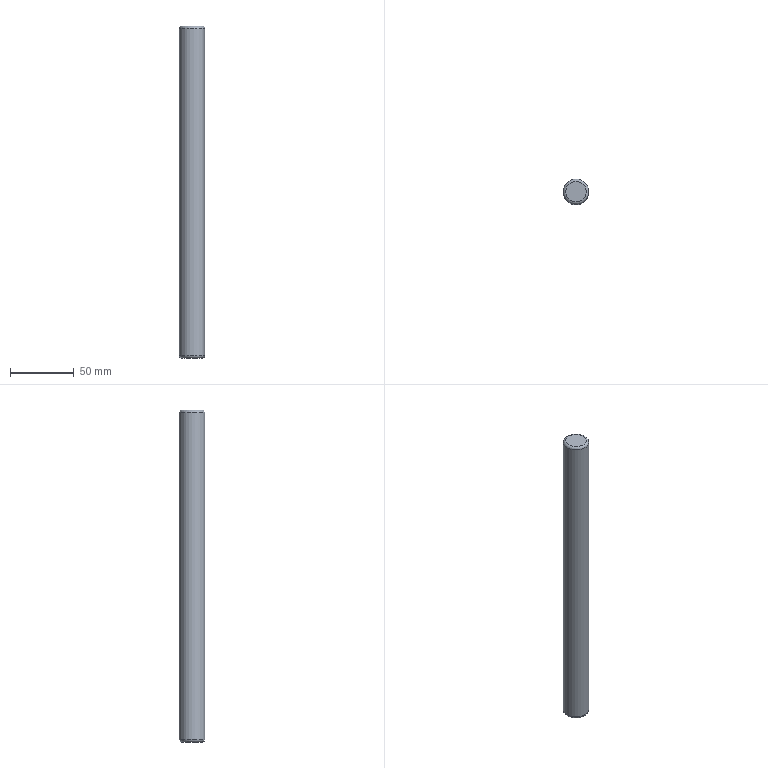Component | NX | CIBIK5 | 1 solid | 5 faces | box 20 x 20 x 260 mm | volume 81578 mm3 | plane 2 | torus 2 | cylinder 1 | commonest cylinder face diameters 20 x1
STEP:
#1=CARTESIAN_POINT('',(0.,0.,0.));
#2=DIRECTION('',(0.,0.,1.));
#3=DIRECTION('',(1.,0.,0.));
#4=AXIS2_PLACEMENT_3D('',#1,#2,#3);
#5=CARTESIAN_POINT('',(-1165.866,976.821,260.));
#6=VERTEX_POINT('',#5);
#7=CARTESIAN_POINT('',(-1155.866,976.821,260.));
#8=DIRECTION('',(0.,0.,-1.));
#9=DIRECTION('',(-1.,0.,0.));
#10=AXIS2_PLACEMENT_3D('',#7,#8,#9);
#11=CIRCLE('',#10,10.);
#12=CARTESIAN_POINT('',(-1155.866,976.821,2.));
#13=DIRECTION('',(0.,0.,1.));
#14=DIRECTION('',(1.,0.,0.));
#15=AXIS2_PLACEMENT_3D('',#12,#13,#14);
#16=CYLINDRICAL_SURFACE('',#15,10.);
#17=CARTESIAN_POINT('',(9.425,258.));
#18=DIRECTION('',(-1.,0.));
#19=VECTOR('',#18,1.);
#20=LINE('',#17,#19);
#21=(GEOMETRIC_REPRESENTATION_CONTEXT(2)PARAMETRIC_REPRESENTATION_CONTEXT()REPRESENTATION_CONTEXT('',''));
#22=DEFINITIONAL_REPRESENTATION('',(#20),#21);
#23=PCURVE('',#16,#22);
#24=CARTESIAN_POINT('',(-1155.866,976.821,260.));
#25=DIRECTION('',(0.,0.,-1.));
#26=DIRECTION('',(-1.,0.,0.));
#27=AXIS2_PLACEMENT_3D('',#24,#25,#26);
#28=TOROIDAL_SURFACE('',#27,8.,2.);
#29=CARTESIAN_POINT('',(0.,6.283));
#30=DIRECTION('',(1.,0.));
#31=VECTOR('',#30,1.);
#32=LINE('',#29,#31);
#33=(GEOMETRIC_REPRESENTATION_CONTEXT(2)PARAMETRIC_REPRESENTATION_CONTEXT()REPRESENTATION_CONTEXT('',''));
#34=DEFINITIONAL_REPRESENTATION('',(#32),#33);
#35=PCURVE('',#28,#34);
#36=SURFACE_CURVE('',#11,(#23,#35),.PCURVE_S1.);
#37=EDGE_CURVE('',#6,#6,#36,.T.);
#38=ORIENTED_EDGE('',*,*,#37,.T.);
#39=CARTESIAN_POINT('',(-1165.866,976.821,4.));
#40=VERTEX_POINT('',#39);
#41=CARTESIAN_POINT('',(-1165.866,976.821,4.));
#42=CARTESIAN_POINT('',(-1165.866,976.821,260.));
#43=B_SPLINE_CURVE_WITH_KNOTS('',1,(#41,#42),.UNSPECIFIED.,.F.,.F.,(2,2),(2.,258.),.PIECEWISE_BEZIER_KNOTS.);
#44=CARTESIAN_POINT('',(3.142,0.));
#45=DIRECTION('',(0.,1.));
#46=VECTOR('',#45,1.);
#47=LINE('',#44,#46);
#48=(GEOMETRIC_REPRESENTATION_CONTEXT(2)PARAMETRIC_REPRESENTATION_CONTEXT()REPRESENTATION_CONTEXT('',''));
#49=DEFINITIONAL_REPRESENTATION('',(#47),#48);
#50=PCURVE('',#16,#49);
#51=CARTESIAN_POINT('',(9.425,0.));
#52=DIRECTION('',(0.,1.));
#53=VECTOR('',#52,1.);
#54=LINE('',#51,#53);
#55=(GEOMETRIC_REPRESENTATION_CONTEXT(2)PARAMETRIC_REPRESENTATION_CONTEXT()REPRESENTATION_CONTEXT('',''));
#56=DEFINITIONAL_REPRESENTATION('',(#54),#55);
#57=PCURVE('',#16,#56);
#58=SEAM_CURVE('',#43,(#50,#57),.PCURVE_S1.);
#59=EDGE_CURVE('',#40,#6,#58,.T.);
#60=ORIENTED_EDGE('',*,*,#59,.F.);
#61=CARTESIAN_POINT('',(-1155.866,976.821,4.));
#62=DIRECTION('',(0.,0.,1.));
#63=DIRECTION('',(-1.,0.,0.));
#64=AXIS2_PLACEMENT_3D('',#61,#62,#63);
#65=CIRCLE('',#64,10.);
#66=CARTESIAN_POINT('',(3.142,2.));
#67=DIRECTION('',(1.,0.));
#68=VECTOR('',#67,1.);
#69=LINE('',#66,#68);
#70=(GEOMETRIC_REPRESENTATION_CONTEXT(2)PARAMETRIC_REPRESENTATION_CONTEXT()REPRESENTATION_CONTEXT('',''));
#71=DEFINITIONAL_REPRESENTATION('',(#69),#70);
#72=PCURVE('',#16,#71);
#73=CARTESIAN_POINT('',(-1155.866,976.821,4.));
#74=DIRECTION('',(0.,0.,-1.));
#75=DIRECTION('',(-1.,0.,0.));
#76=AXIS2_PLACEMENT_3D('',#73,#74,#75);
#77=TOROIDAL_SURFACE('',#76,8.,2.);
#78=CARTESIAN_POINT('',(6.283,6.283));
#79=DIRECTION('',(-1.,0.));
#80=VECTOR('',#79,1.);
#81=LINE('',#78,#80);
#82=(GEOMETRIC_REPRESENTATION_CONTEXT(2)PARAMETRIC_REPRESENTATION_CONTEXT()REPRESENTATION_CONTEXT('',''));
#83=DEFINITIONAL_REPRESENTATION('',(#81),#82);
#84=PCURVE('',#77,#83);
#85=SURFACE_CURVE('',#65,(#72,#84),.PCURVE_S1.);
#86=EDGE_CURVE('',#40,#40,#85,.T.);
#87=ORIENTED_EDGE('',*,*,#86,.T.);
#88=ORIENTED_EDGE('',*,*,#59,.T.);
#89=EDGE_LOOP('',(#38,#60,#87,#88));
#90=FACE_BOUND('',#89,.T.);
#91=ADVANCED_FACE('',(#90),#16,.T.);
#92=CARTESIAN_POINT('',(-1163.866,976.821,2.));
#93=VERTEX_POINT('',#92);
#94=CARTESIAN_POINT('',(-1155.866,976.821,2.));
#95=DIRECTION('',(0.,0.,-1.));
#96=DIRECTION('',(-1.,0.,0.));
#97=AXIS2_PLACEMENT_3D('',#94,#95,#96);
#98=CIRCLE('',#97,8.);
#99=CARTESIAN_POINT('',(-1155.866,976.821,2.));
#100=DIRECTION('',(0.,0.,-1.));
#101=DIRECTION('',(-1.,0.,0.));
#102=AXIS2_PLACEMENT_3D('',#99,#100,#101);
#103=PLANE('',#102);
#104=CARTESIAN_POINT('',(0.,0.));
#105=DIRECTION('',(1.,0.));
#106=AXIS2_PLACEMENT_2D('',#104,#105);
#107=CIRCLE('',#106,8.);
#108=(GEOMETRIC_REPRESENTATION_CONTEXT(2)PARAMETRIC_REPRESENTATION_CONTEXT()REPRESENTATION_CONTEXT('',''));
#109=DEFINITIONAL_REPRESENTATION('',(#107),#108);
#110=PCURVE('',#103,#109);
#111=CARTESIAN_POINT('',(0.,7.854));
#112=DIRECTION('',(1.,0.));
#113=VECTOR('',#112,1.);
#114=LINE('',#111,#113);
#115=(GEOMETRIC_REPRESENTATION_CONTEXT(2)PARAMETRIC_REPRESENTATION_CONTEXT()REPRESENTATION_CONTEXT('',''));
#116=DEFINITIONAL_REPRESENTATION('',(#114),#115);
#117=PCURVE('',#77,#116);
#118=SURFACE_CURVE('',#98,(#110,#117),.PCURVE_S1.);
#119=EDGE_CURVE('',#93,#93,#118,.T.);
#120=ORIENTED_EDGE('',*,*,#119,.T.);
#121=EDGE_LOOP('',(#120));
#122=FACE_BOUND('',#121,.T.);
#123=ADVANCED_FACE('',(#122),#103,.T.);
#124=CARTESIAN_POINT('',(-1163.866,976.821,262.));
#125=VERTEX_POINT('',#124);
#126=CARTESIAN_POINT('',(-1155.866,976.821,262.));
#127=DIRECTION('',(0.,0.,1.));
#128=DIRECTION('',(-1.,0.,0.));
#129=AXIS2_PLACEMENT_3D('',#126,#127,#128);
#130=CIRCLE('',#129,8.);
#131=CARTESIAN_POINT('',(-1155.866,976.821,262.));
#132=DIRECTION('',(0.,0.,-1.));
#133=DIRECTION('',(-1.,0.,0.));
#134=AXIS2_PLACEMENT_3D('',#131,#132,#133);
#135=PLANE('',#134);
#136=CARTESIAN_POINT('',(8.,0.));
#137=CARTESIAN_POINT('',(8.,-13.856));
#138=CARTESIAN_POINT('',(-4.,-6.928));
#139=CARTESIAN_POINT('',(-16.,-0.));
#140=CARTESIAN_POINT('',(-4.,6.928));
#141=CARTESIAN_POINT('',(8.,13.856));
#142=CARTESIAN_POINT('',(8.,0.));
#143=(BOUNDED_CURVE()B_SPLINE_CURVE(2,(#136,#137,#138,#139,#140,#141,#142),.UNSPECIFIED.,.T.,.F.)B_SPLINE_CURVE_WITH_KNOTS((1,2,2,2,2,1),(-2.094,0.,2.094,4.189,6.283,8.378),.UNSPECIFIED.)CURVE()GEOMETRIC_REPRESENTATION_ITEM()RATIONAL_B_SPLINE_CURVE((1.,0.5,1.,0.5,1.,0.5,1.))REPRESENTATION_ITEM(''));
#144=(GEOMETRIC_REPRESENTATION_CONTEXT(2)PARAMETRIC_REPRESENTATION_CONTEXT()REPRESENTATION_CONTEXT('',''));
#145=DEFINITIONAL_REPRESENTATION('',(#143),#144);
#146=PCURVE('',#135,#145);
#147=CARTESIAN_POINT('',(6.283,4.712));
#148=DIRECTION('',(-1.,0.));
#149=VECTOR('',#148,1.);
#150=LINE('',#147,#149);
#151=(GEOMETRIC_REPRESENTATION_CONTEXT(2)PARAMETRIC_REPRESENTATION_CONTEXT()REPRESENTATION_CONTEXT('',''));
#152=DEFINITIONAL_REPRESENTATION('',(#150),#151);
#153=PCURVE('',#28,#152);
#154=SURFACE_CURVE('',#130,(#146,#153),.PCURVE_S1.);
#155=EDGE_CURVE('',#125,#125,#154,.T.);
#156=ORIENTED_EDGE('',*,*,#155,.T.);
#157=EDGE_LOOP('',(#156));
#158=FACE_BOUND('',#157,.T.);
#159=ADVANCED_FACE('',(#158),#135,.F.);
#160=ORIENTED_EDGE('',*,*,#155,.F.);
#161=CARTESIAN_POINT('',(-1163.866,976.821,262.));
#162=CARTESIAN_POINT('',(-1164.401,976.821,262.));
#163=CARTESIAN_POINT('',(-1164.922,976.821,261.83));
#164=CARTESIAN_POINT('',(-1165.37,976.821,261.504));
#165=CARTESIAN_POINT('',(-1165.696,976.821,261.055));
#166=CARTESIAN_POINT('',(-1165.866,976.821,260.535));
#167=CARTESIAN_POINT('',(-1165.866,976.821,260.));
#168=(BOUNDED_CURVE()B_SPLINE_CURVE(6,(#161,#162,#163,#164,#165,#166,#167),.UNSPECIFIED.,.F.,.F.)B_SPLINE_CURVE_WITH_KNOTS((7,7),(4.712,6.283),.PIECEWISE_BEZIER_KNOTS.)CURVE()GEOMETRIC_REPRESENTATION_ITEM()RATIONAL_B_SPLINE_CURVE((1.031,1.01,0.9979,0.994,0.9979,1.01,1.031))REPRESENTATION_ITEM(''));
#169=CARTESIAN_POINT('',(6.283,0.));
#170=DIRECTION('',(0.,1.));
#171=VECTOR('',#170,1.);
#172=LINE('',#169,#171);
#173=(GEOMETRIC_REPRESENTATION_CONTEXT(2)PARAMETRIC_REPRESENTATION_CONTEXT()REPRESENTATION_CONTEXT('',''));
#174=DEFINITIONAL_REPRESENTATION('',(#172),#173);
#175=PCURVE('',#28,#174);
#176=CARTESIAN_POINT('',(0.,0.));
#177=DIRECTION('',(0.,1.));
#178=VECTOR('',#177,1.);
#179=LINE('',#176,#178);
#180=(GEOMETRIC_REPRESENTATION_CONTEXT(2)PARAMETRIC_REPRESENTATION_CONTEXT()REPRESENTATION_CONTEXT('',''));
#181=DEFINITIONAL_REPRESENTATION('',(#179),#180);
#182=PCURVE('',#28,#181);
#183=SEAM_CURVE('',#168,(#175,#182),.PCURVE_S1.);
#184=EDGE_CURVE('',#125,#6,#183,.T.);
#185=ORIENTED_EDGE('',*,*,#184,.T.);
#186=ORIENTED_EDGE('',*,*,#37,.F.);
#187=ORIENTED_EDGE('',*,*,#184,.F.);
#188=EDGE_LOOP('',(#160,#185,#186,#187));
#189=FACE_BOUND('',#188,.T.);
#190=ADVANCED_FACE('',(#189),#28,.T.);
#191=ORIENTED_EDGE('',*,*,#86,.F.);
#192=CARTESIAN_POINT('',(-1165.866,976.821,4.));
#193=CARTESIAN_POINT('',(-1165.866,976.821,3.465));
#194=CARTESIAN_POINT('',(-1165.696,976.821,2.945));
#195=CARTESIAN_POINT('',(-1165.37,976.821,2.496));
#196=CARTESIAN_POINT('',(-1164.922,976.821,2.17));
#197=CARTESIAN_POINT('',(-1164.401,976.821,2.));
#198=CARTESIAN_POINT('',(-1163.866,976.821,2.));
#199=(BOUNDED_CURVE()B_SPLINE_CURVE(6,(#192,#193,#194,#195,#196,#197,#198),.UNSPECIFIED.,.F.,.F.)B_SPLINE_CURVE_WITH_KNOTS((7,7),(0.,1.571),.PIECEWISE_BEZIER_KNOTS.)CURVE()GEOMETRIC_REPRESENTATION_ITEM()RATIONAL_B_SPLINE_CURVE((1.031,1.01,0.9979,0.994,0.9979,1.01,1.031))REPRESENTATION_ITEM(''));
#200=CARTESIAN_POINT('',(6.283,6.283));
#201=DIRECTION('',(0.,1.));
#202=VECTOR('',#201,1.);
#203=LINE('',#200,#202);
#204=(GEOMETRIC_REPRESENTATION_CONTEXT(2)PARAMETRIC_REPRESENTATION_CONTEXT()REPRESENTATION_CONTEXT('',''));
#205=DEFINITIONAL_REPRESENTATION('',(#203),#204);
#206=PCURVE('',#77,#205);
#207=CARTESIAN_POINT('',(0.,6.283));
#208=DIRECTION('',(0.,1.));
#209=VECTOR('',#208,1.);
#210=LINE('',#207,#209);
#211=(GEOMETRIC_REPRESENTATION_CONTEXT(2)PARAMETRIC_REPRESENTATION_CONTEXT()REPRESENTATION_CONTEXT('',''));
#212=DEFINITIONAL_REPRESENTATION('',(#210),#211);
#213=PCURVE('',#77,#212);
#214=SEAM_CURVE('',#199,(#206,#213),.PCURVE_S1.);
#215=EDGE_CURVE('',#40,#93,#214,.T.);
#216=ORIENTED_EDGE('',*,*,#215,.T.);
#217=ORIENTED_EDGE('',*,*,#119,.F.);
#218=ORIENTED_EDGE('',*,*,#215,.F.);
#219=EDGE_LOOP('',(#191,#216,#217,#218));
#220=FACE_BOUND('',#219,.T.);
#221=ADVANCED_FACE('',(#220),#77,.T.);
#222=CLOSED_SHELL('',(#91,#123,#159,#190,#221));
#223=MANIFOLD_SOLID_BREP('',#222);
#224=(LENGTH_UNIT()NAMED_UNIT(*)SI_UNIT(.MILLI.,.METRE.));
#225=UNCERTAINTY_MEASURE_WITH_UNIT(LENGTH_MEASURE(0.00001),#224,'','');
#226=(NAMED_UNIT(*)PLANE_ANGLE_UNIT()SI_UNIT($,.RADIAN.));
#227=(NAMED_UNIT(*)SI_UNIT($,.STERADIAN.)SOLID_ANGLE_UNIT());
#228=(GEOMETRIC_REPRESENTATION_CONTEXT(3)GLOBAL_UNCERTAINTY_ASSIGNED_CONTEXT((#225))GLOBAL_UNIT_ASSIGNED_CONTEXT((#224,#226,#227))REPRESENTATION_CONTEXT('',''));
#229=ADVANCED_BREP_SHAPE_REPRESENTATION('',(#4,#223),#228);